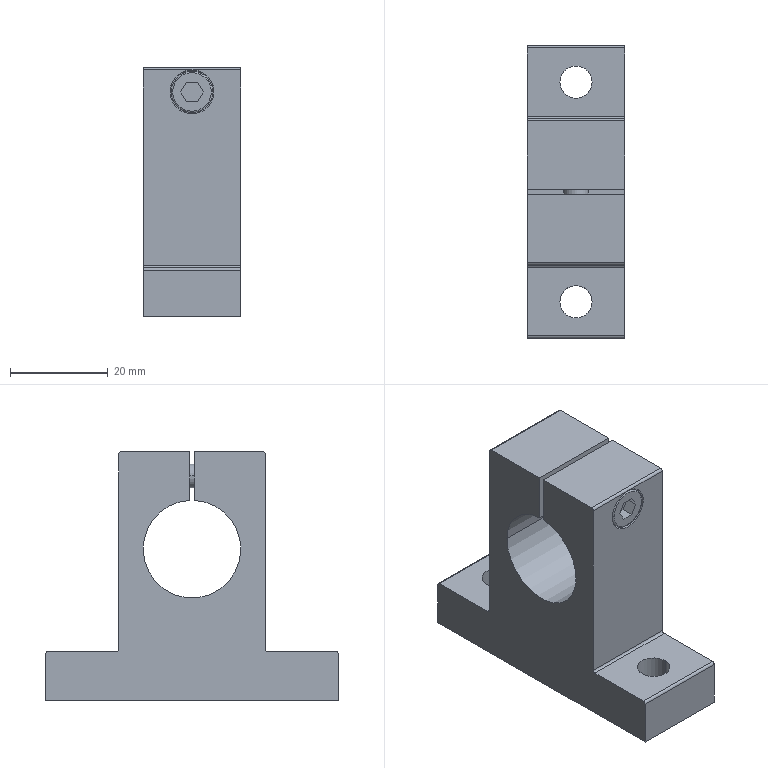Component | SolidWorks | GFF01-D20-2 | 1 solid | 43 faces | volume 29381 mm3 | plane 22 | cylinder 19 | spline 2 | commonest cylinder face diameters 1 x6 6.6 x4 20 x3 5 x2 8.5 x2 9 x2